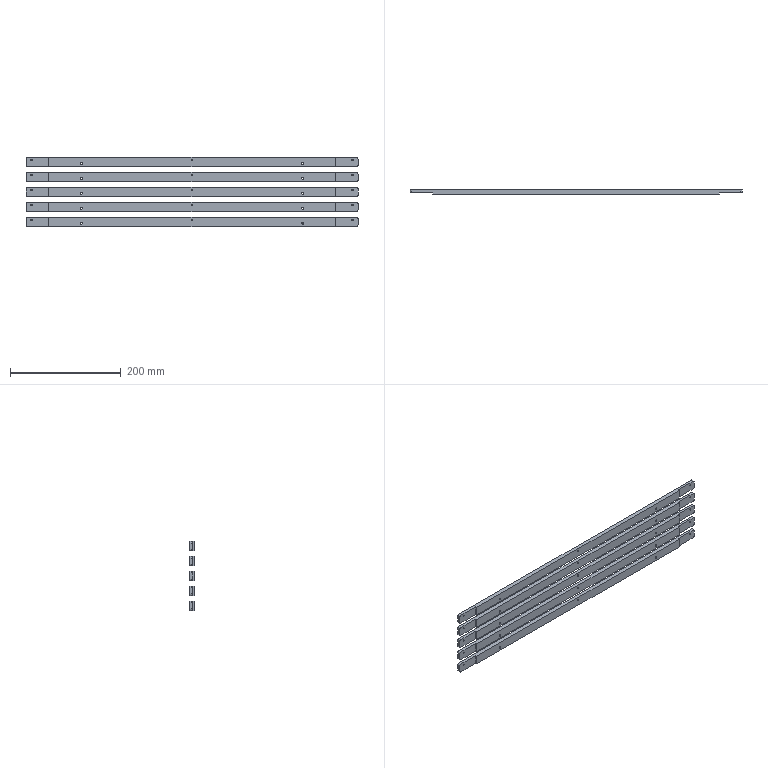CAM job | Mastercam | mm | 10 operations | part box 600 x 7.5 x 125
1. Facing | 24 - 100 平铣刀
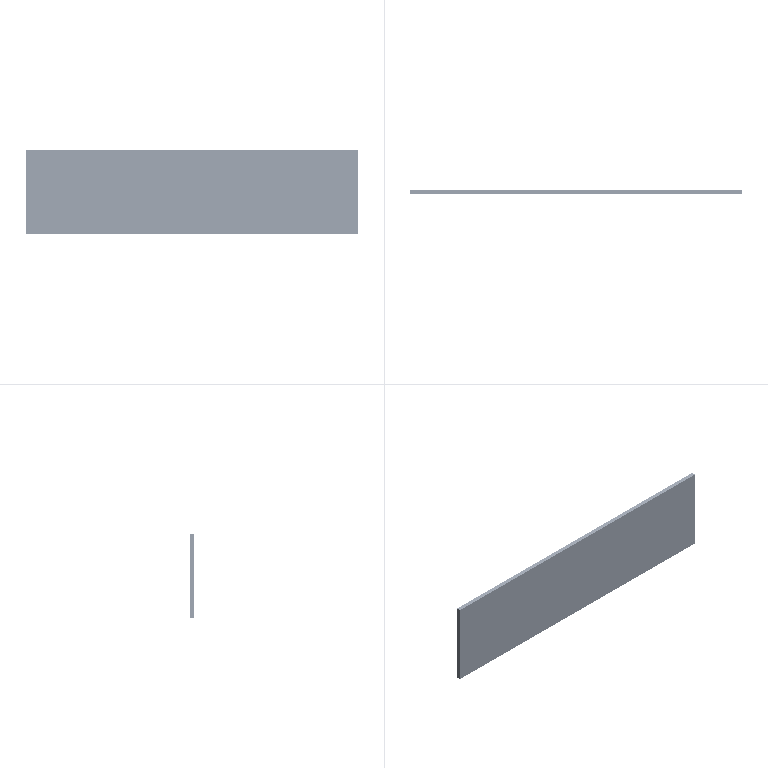2. Contour (Ramp) | 10 - 10 平铣刀
3. Contour (2D) | 10 - 10 平铣刀
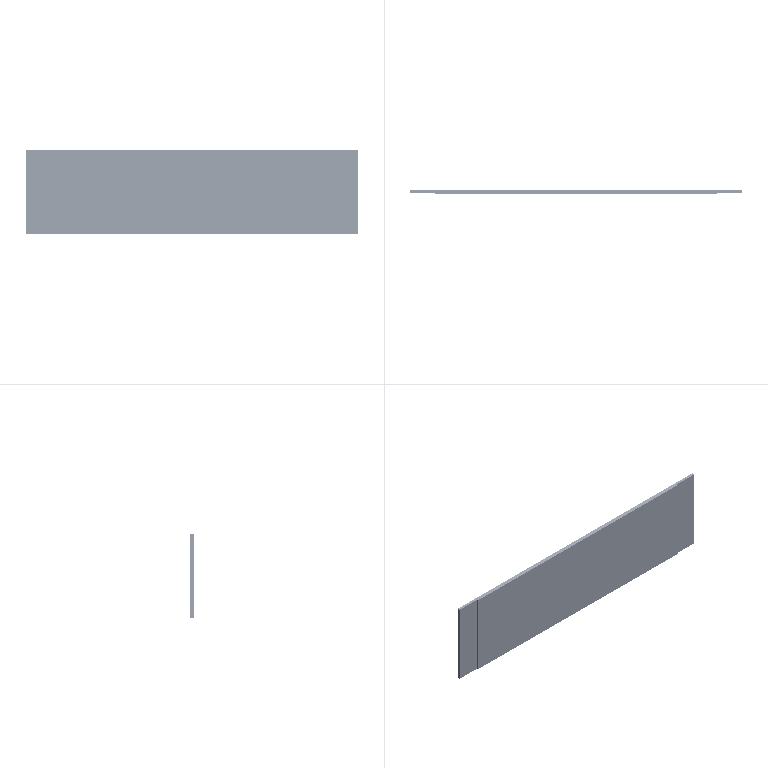4. Contour (Ramp) | 10 - 10 平铣刀
5. Contour (2D) | 10 - 10 平铣刀
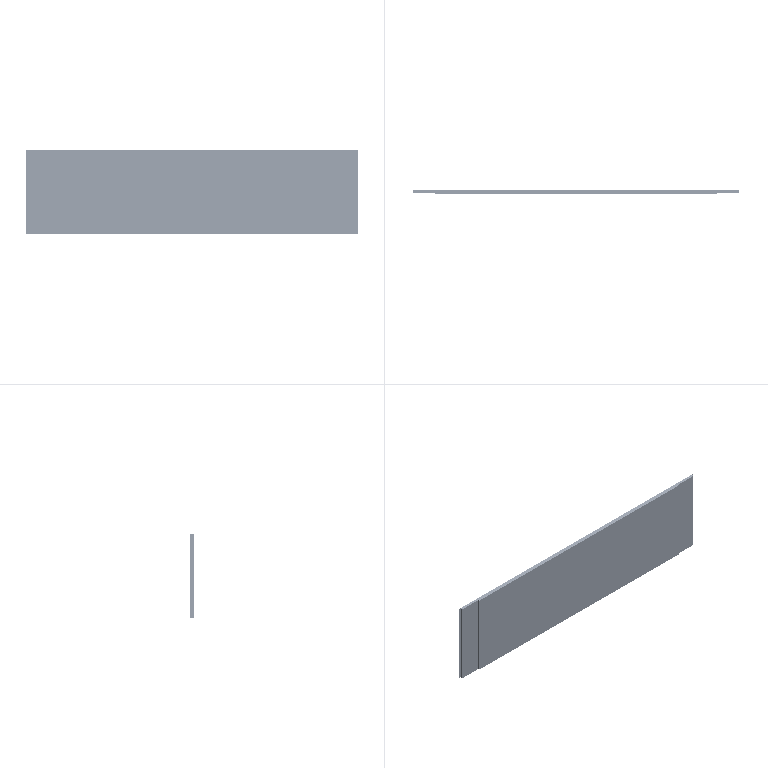6. Contour (Ramp) | 4 - 4 平铣刀
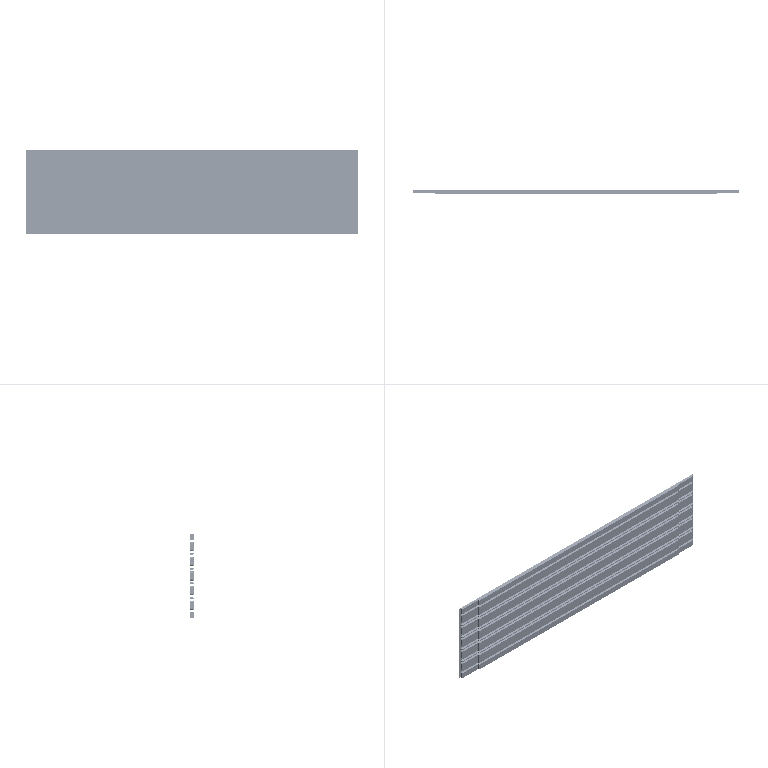7. Drill/Counterbore | 7 - 4 倒角刀
8. Contour (2D chamfer) | 7 - 4 倒角刀
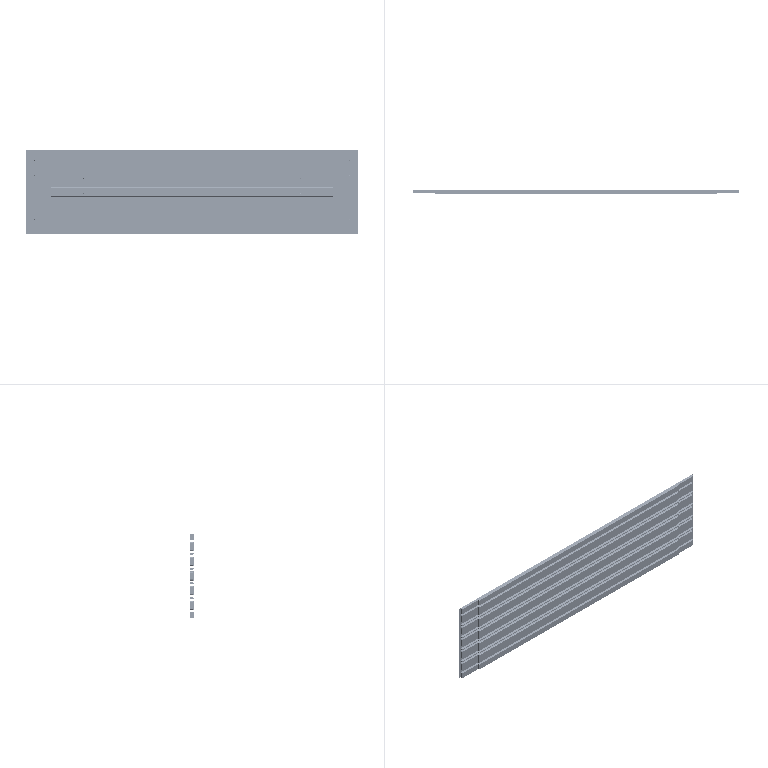9. Contour (2D chamfer) | 7 - 4 倒角刀
10. Contour (Ramp) | 3 - 3 平铣刀